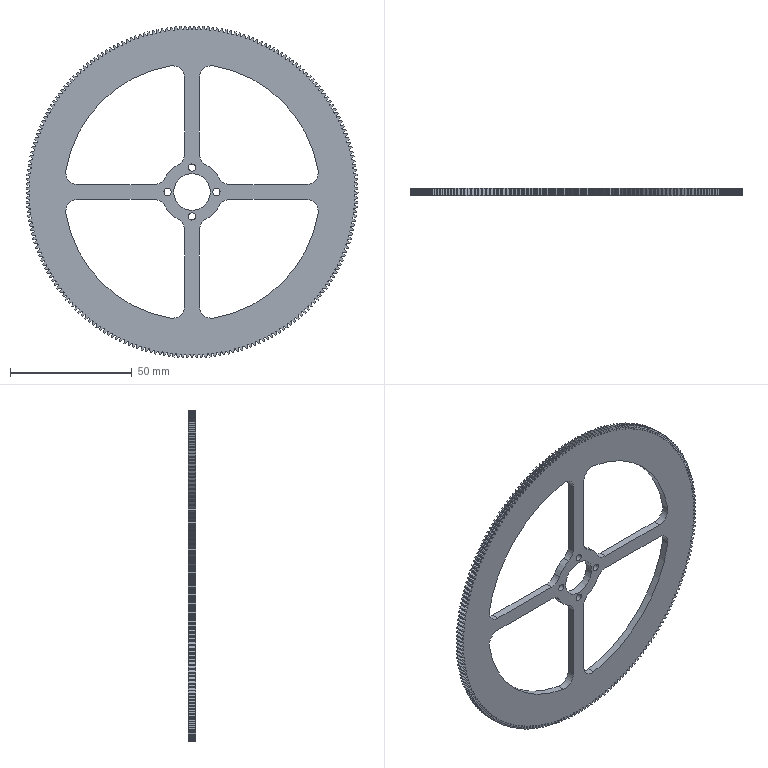Component | NX | 225_GEAR | 1 solid | 1389 faces | volume 20883 mm3 | other 1125 | cylinder 254 | plane 10 | commonest cylinder face diameters 133.5 x225 10 x16 105 x4 25 x4 3 x4 15 x1